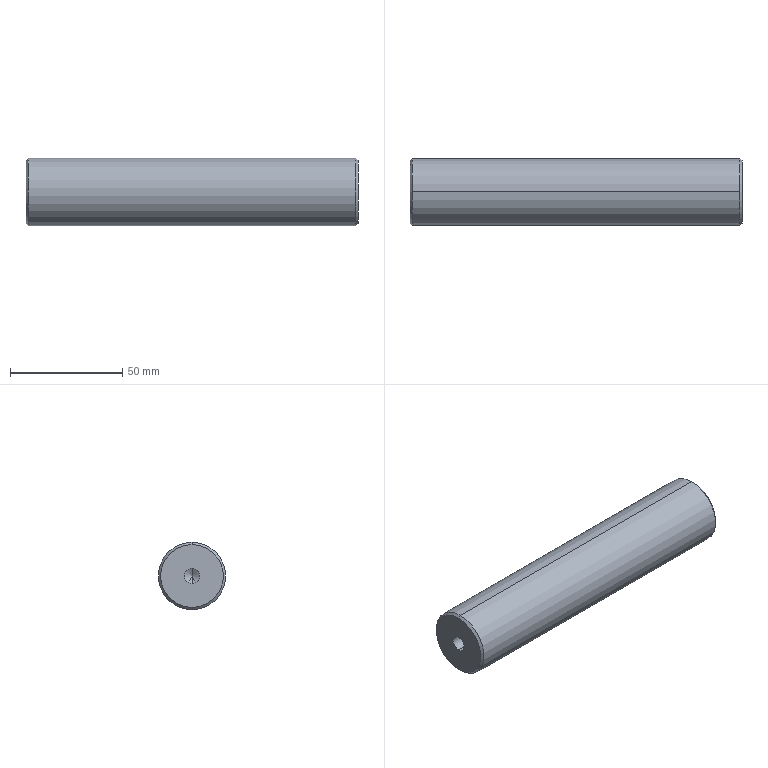Component | SolidWorks | GuideMechanism-1_ConnectingRod-1 | 1 solid | 16 faces | box 148 x 30 x 30 mm | volume 103039 mm3 | cone 8 | cylinder 6 | plane 2 | commonest cylinder face diameters 6.8 x4 30 x2
build123d program:
from build123d import *

# Parameters (mm, degrees)
SKETCH1_R           = 15
BOSS_EXTRUDE1_DEPTH = 74
CHAMFER1_SIZE       = 1


with BuildPart() as part:
    # Sketch1 → Boss-Extrude1 (new, symmetric)
    with BuildSketch(Plane(origin=(0, 0, 0), x_dir=(0, 0, -1), z_dir=(1, 0, 0))):
        Circle(SKETCH1_R)
    extrude(amount=BOSS_EXTRUDE1_DEPTH, both=True)

    # Sketch3 → M8 Tapped Hole1 (revolve, cut)
    with BuildSketch(Plane(origin=(74, 0, 0), x_dir=(0, 0, -1), z_dir=(0, 1, 0))):
        Polygon((0, 0), (0, 21.793), (3.4, 19.75), (3.4, 0), align=None)
    m8_tapped_hole1 = revolve(axis=Axis((80.35, 0, 0), (-1, 0, 0)), mode=Mode.SUBTRACT)

    # Mirror1: M8 Tapped Hole1 across plane
    add(m8_tapped_hole1.mirror(Plane(origin=(0, 0, 0), x_dir=(0, 0, 1), z_dir=(1, 0, 0))), mode=Mode.SUBTRACT)

    # Chamfer1
    chamfer1_edges = [part.edges().sort_by_distance(p)[0] for p in [
        (-74, 0, 15),
        (74, 0, 15),
    ]]
    chamfer(chamfer1_edges, length=CHAMFER1_SIZE)


solid = part.part

# Placed as in the assembly
solid = solid.moved(Location((-439.272, -518.766, 1326.5), (0, 0, 0)))
STEP:
#1=COLOUR_RGB('',0.7922,0.8196,0.9333);
#2=FILL_AREA_STYLE_COLOUR('',#1);
#3=FILL_AREA_STYLE('',(#2));
#4=SURFACE_STYLE_FILL_AREA(#3);
#5=SURFACE_SIDE_STYLE('',(#4));
#6=SURFACE_STYLE_USAGE(.BOTH.,#5);
#7=PRESENTATION_STYLE_ASSIGNMENT((#6));
#8=CARTESIAN_POINT('',(-20.208,-20.424,52.776));
#9=VERTEX_POINT('',#8);
#10=CARTESIAN_POINT('',(-20.208,-20.424,51.673));
#11=VERTEX_POINT('',#10);
#12=CARTESIAN_POINT('',(-20.208,-20.424,52.224));
#13=DIRECTION('',(-1.,0.,0.));
#14=DIRECTION('',(0.,0.,-1.));
#15=AXIS2_PLACEMENT_3D('',#12,#13,#14);
#16=CIRCLE('',#15,0.5512);
#17=EDGE_CURVE('',#9,#11,#16,.T.);
#18=ORIENTED_EDGE('',*,*,#17,.F.);
#19=CARTESIAN_POINT('',(-20.168,-20.424,52.815));
#20=VERTEX_POINT('',#19);
#21=CARTESIAN_POINT('',(-20.168,-20.424,52.815));
#22=DIRECTION('',(0.7071,0.,0.7071));
#23=VECTOR('',#22,39.37);
#24=LINE('',#21,#23);
#25=EDGE_CURVE('',#9,#20,#24,.T.);
#26=ORIENTED_EDGE('',*,*,#25,.T.);
#27=CARTESIAN_POINT('',(-20.168,-20.424,51.634));
#28=VERTEX_POINT('',#27);
#29=CARTESIAN_POINT('',(-20.168,-20.424,52.224));
#30=DIRECTION('',(1.,0.,0.));
#31=DIRECTION('',(0.,0.,-1.));
#32=AXIS2_PLACEMENT_3D('',#29,#30,#31);
#33=CIRCLE('',#32,0.5906);
#34=EDGE_CURVE('',#28,#20,#33,.T.);
#35=ORIENTED_EDGE('',*,*,#34,.F.);
#36=CARTESIAN_POINT('',(-20.168,-20.424,51.634));
#37=DIRECTION('',(0.7071,0.,-0.7071));
#38=VECTOR('',#37,39.37);
#39=LINE('',#36,#38);
#40=EDGE_CURVE('',#11,#28,#39,.T.);
#41=ORIENTED_EDGE('',*,*,#40,.F.);
#42=EDGE_LOOP('',(#18,#26,#35,#41));
#43=FACE_OUTER_BOUND('',#42,.T.);
#44=CARTESIAN_POINT('',(-20.168,-20.424,52.224));
#45=DIRECTION('',(1.,0.,0.));
#46=DIRECTION('',(0.,0.,-1.));
#47=AXIS2_PLACEMENT_3D('',#44,#45,#46);
#48=CONICAL_SURFACE('',#47,0.5906,0.7854);
#49=ADVANCED_FACE('',(#43),#48,.T.);
#50=CARTESIAN_POINT('',(-14.381,-20.424,51.673));
#51=VERTEX_POINT('',#50);
#52=CARTESIAN_POINT('',(-14.381,-20.424,52.776));
#53=VERTEX_POINT('',#52);
#54=CARTESIAN_POINT('',(-14.381,-20.424,52.224));
#55=DIRECTION('',(1.,0.,0.));
#56=DIRECTION('',(0.,0.,-1.));
#57=AXIS2_PLACEMENT_3D('',#54,#55,#56);
#58=CIRCLE('',#57,0.5512);
#59=EDGE_CURVE('',#51,#53,#58,.T.);
#60=ORIENTED_EDGE('',*,*,#59,.F.);
#61=CARTESIAN_POINT('',(-14.42,-20.424,51.634));
#62=VERTEX_POINT('',#61);
#63=CARTESIAN_POINT('',(-14.381,-20.424,51.673));
#64=DIRECTION('',(-0.7071,0.,-0.7071));
#65=VECTOR('',#64,39.37);
#66=LINE('',#63,#65);
#67=EDGE_CURVE('',#51,#62,#66,.T.);
#68=ORIENTED_EDGE('',*,*,#67,.T.);
#69=CARTESIAN_POINT('',(-14.42,-20.424,52.815));
#70=VERTEX_POINT('',#69);
#71=CARTESIAN_POINT('',(-14.42,-20.424,52.224));
#72=DIRECTION('',(-1.,0.,0.));
#73=DIRECTION('',(0.,0.,-1.));
#74=AXIS2_PLACEMENT_3D('',#71,#72,#73);
#75=CIRCLE('',#74,0.5906);
#76=EDGE_CURVE('',#70,#62,#75,.T.);
#77=ORIENTED_EDGE('',*,*,#76,.F.);
#78=CARTESIAN_POINT('',(-14.381,-20.424,52.776));
#79=DIRECTION('',(-0.7071,0.,0.7071));
#80=VECTOR('',#79,39.37);
#81=LINE('',#78,#80);
#82=EDGE_CURVE('',#53,#70,#81,.T.);
#83=ORIENTED_EDGE('',*,*,#82,.F.);
#84=EDGE_LOOP('',(#60,#68,#77,#83));
#85=FACE_OUTER_BOUND('',#84,.T.);
#86=CARTESIAN_POINT('',(-14.381,-20.424,52.224));
#87=DIRECTION('',(-1.,0.,0.));
#88=DIRECTION('',(0.,0.,1.));
#89=AXIS2_PLACEMENT_3D('',#86,#87,#88);
#90=CONICAL_SURFACE('',#89,0.5512,0.7854);
#91=ADVANCED_FACE('',(#85),#90,.T.);
#92=CARTESIAN_POINT('',(-19.43,-20.424,52.091));
#93=VERTEX_POINT('',#92);
#94=CARTESIAN_POINT('',(-19.43,-20.424,52.358));
#95=VERTEX_POINT('',#94);
#96=CARTESIAN_POINT('',(-19.43,-20.424,52.224));
#97=DIRECTION('',(-1.,0.,0.));
#98=DIRECTION('',(0.,0.,1.));
#99=AXIS2_PLACEMENT_3D('',#96,#97,#98);
#100=CIRCLE('',#99,0.1339);
#101=EDGE_CURVE('',#93,#95,#100,.T.);
#102=ORIENTED_EDGE('',*,*,#101,.F.);
#103=CARTESIAN_POINT('',(-20.208,-20.424,52.091));
#104=VERTEX_POINT('',#103);
#105=CARTESIAN_POINT('',(-20.208,-20.424,52.091));
#106=DIRECTION('',(-1.,0.,0.));
#107=VECTOR('',#106,39.37);
#108=LINE('',#105,#107);
#109=EDGE_CURVE('',#93,#104,#108,.T.);
#110=ORIENTED_EDGE('',*,*,#109,.T.);
#111=CARTESIAN_POINT('',(-20.208,-20.424,52.358));
#112=VERTEX_POINT('',#111);
#113=CARTESIAN_POINT('',(-20.208,-20.424,52.224));
#114=DIRECTION('',(-1.,0.,0.));
#115=DIRECTION('',(0.,0.,1.));
#116=AXIS2_PLACEMENT_3D('',#113,#114,#115);
#117=CIRCLE('',#116,0.1339);
#118=EDGE_CURVE('',#104,#112,#117,.T.);
#119=ORIENTED_EDGE('',*,*,#118,.T.);
#120=CARTESIAN_POINT('',(-20.208,-20.424,52.358));
#121=DIRECTION('',(-1.,0.,0.));
#122=VECTOR('',#121,39.37);
#123=LINE('',#120,#122);
#124=EDGE_CURVE('',#95,#112,#123,.T.);
#125=ORIENTED_EDGE('',*,*,#124,.F.);
#126=EDGE_LOOP('',(#102,#110,#119,#125));
#127=FACE_OUTER_BOUND('',#126,.T.);
#128=CARTESIAN_POINT('',(-20.208,-20.424,52.224));
#129=DIRECTION('',(-1.,0.,0.));
#130=DIRECTION('',(0.,0.,1.));
#131=AXIS2_PLACEMENT_3D('',#128,#129,#130);
#132=CYLINDRICAL_SURFACE('',#131,0.1339);
#133=ADVANCED_FACE('',(#127),#132,.F.);
#134=CARTESIAN_POINT('',(-19.35,-20.424,52.224));
#135=VERTEX_POINT('',#134);
#136=CARTESIAN_POINT('',(-19.43,-20.424,52.358));
#137=DIRECTION('',(-0.515,0.,0.8572));
#138=VECTOR('',#137,39.37);
#139=LINE('',#136,#138);
#140=EDGE_CURVE('',#135,#95,#139,.T.);
#141=ORIENTED_EDGE('',*,*,#140,.F.);
#142=CARTESIAN_POINT('',(-19.43,-20.424,52.091));
#143=DIRECTION('',(-0.515,0.,-0.8572));
#144=VECTOR('',#143,39.37);
#145=LINE('',#142,#144);
#146=EDGE_CURVE('',#135,#93,#145,.T.);
#147=ORIENTED_EDGE('',*,*,#146,.T.);
#148=ORIENTED_EDGE('',*,*,#101,.T.);
#149=EDGE_LOOP('',(#141,#147,#148));
#150=FACE_OUTER_BOUND('',#149,.T.);
#151=CARTESIAN_POINT('',(-19.43,-20.424,52.224));
#152=DIRECTION('',(-1.,0.,0.));
#153=DIRECTION('',(0.,0.,1.));
#154=AXIS2_PLACEMENT_3D('',#151,#152,#153);
#155=CONICAL_SURFACE('',#154,0.1339,1.03);
#156=ADVANCED_FACE('',(#150),#155,.F.);
#157=CARTESIAN_POINT('',(-15.158,-20.424,52.358));
#158=VERTEX_POINT('',#157);
#159=CARTESIAN_POINT('',(-15.158,-20.424,52.091));
#160=VERTEX_POINT('',#159);
#161=CARTESIAN_POINT('',(-15.158,-20.424,52.224));
#162=DIRECTION('',(1.,0.,0.));
#163=DIRECTION('',(0.,0.,-1.));
#164=AXIS2_PLACEMENT_3D('',#161,#162,#163);
#165=CIRCLE('',#164,0.1339);
#166=EDGE_CURVE('',#158,#160,#165,.T.);
#167=ORIENTED_EDGE('',*,*,#166,.F.);
#168=CARTESIAN_POINT('',(-14.381,-20.424,52.358));
#169=VERTEX_POINT('',#168);
#170=CARTESIAN_POINT('',(-14.381,-20.424,52.358));
#171=DIRECTION('',(1.,0.,0.));
#172=VECTOR('',#171,39.37);
#173=LINE('',#170,#172);
#174=EDGE_CURVE('',#158,#169,#173,.T.);
#175=ORIENTED_EDGE('',*,*,#174,.T.);
#176=CARTESIAN_POINT('',(-14.381,-20.424,52.091));
#177=VERTEX_POINT('',#176);
#178=CARTESIAN_POINT('',(-14.381,-20.424,52.224));
#179=DIRECTION('',(1.,0.,0.));
#180=DIRECTION('',(0.,0.,-1.));
#181=AXIS2_PLACEMENT_3D('',#178,#179,#180);
#182=CIRCLE('',#181,0.1339);
#183=EDGE_CURVE('',#169,#177,#182,.T.);
#184=ORIENTED_EDGE('',*,*,#183,.T.);
#185=CARTESIAN_POINT('',(-14.381,-20.424,52.091));
#186=DIRECTION('',(1.,0.,0.));
#187=VECTOR('',#186,39.37);
#188=LINE('',#185,#187);
#189=EDGE_CURVE('',#160,#177,#188,.T.);
#190=ORIENTED_EDGE('',*,*,#189,.F.);
#191=EDGE_LOOP('',(#167,#175,#184,#190));
#192=FACE_OUTER_BOUND('',#191,.T.);
#193=CARTESIAN_POINT('',(-14.381,-20.424,52.224));
#194=DIRECTION('',(1.,0.,0.));
#195=DIRECTION('',(0.,0.,-1.));
#196=AXIS2_PLACEMENT_3D('',#193,#194,#195);
#197=CYLINDRICAL_SURFACE('',#196,0.1339);
#198=ADVANCED_FACE('',(#192),#197,.F.);
#199=CARTESIAN_POINT('',(-15.239,-20.424,52.224));
#200=VERTEX_POINT('',#199);
#201=CARTESIAN_POINT('',(-15.158,-20.424,52.091));
#202=DIRECTION('',(0.515,0.,-0.8572));
#203=VECTOR('',#202,39.37);
#204=LINE('',#201,#203);
#205=EDGE_CURVE('',#200,#160,#204,.T.);
#206=ORIENTED_EDGE('',*,*,#205,.F.);
#207=CARTESIAN_POINT('',(-15.158,-20.424,52.358));
#208=DIRECTION('',(0.515,0.,0.8572));
#209=VECTOR('',#208,39.37);
#210=LINE('',#207,#209);
#211=EDGE_CURVE('',#200,#158,#210,.T.);
#212=ORIENTED_EDGE('',*,*,#211,.T.);
#213=ORIENTED_EDGE('',*,*,#166,.T.);
#214=EDGE_LOOP('',(#206,#212,#213));
#215=FACE_OUTER_BOUND('',#214,.T.);
#216=CARTESIAN_POINT('',(-15.158,-20.424,52.224));
#217=DIRECTION('',(1.,0.,0.));
#218=DIRECTION('',(0.,0.,-1.));
#219=AXIS2_PLACEMENT_3D('',#216,#217,#218);
#220=CONICAL_SURFACE('',#219,0.1339,1.03);
#221=ADVANCED_FACE('',(#215),#220,.F.);
#222=ORIENTED_EDGE('',*,*,#76,.T.);
#223=CARTESIAN_POINT('',(-14.381,-20.424,51.634));
#224=DIRECTION('',(-1.,0.,0.));
#225=VECTOR('',#224,39.37);
#226=LINE('',#223,#225);
#227=EDGE_CURVE('',#62,#28,#226,.T.);
#228=ORIENTED_EDGE('',*,*,#227,.T.);
#229=ORIENTED_EDGE('',*,*,#34,.T.);
#230=CARTESIAN_POINT('',(-14.381,-20.424,52.815));
#231=DIRECTION('',(-1.,0.,0.));
#232=VECTOR('',#231,39.37);
#233=LINE('',#230,#232);
#234=EDGE_CURVE('',#70,#20,#233,.T.);
#235=ORIENTED_EDGE('',*,*,#234,.F.);
#236=EDGE_LOOP('',(#222,#228,#229,#235));
#237=FACE_OUTER_BOUND('',#236,.T.);
#238=CARTESIAN_POINT('',(-14.381,-20.424,52.224));
#239=DIRECTION('',(-1.,0.,0.));
#240=DIRECTION('',(0.,0.,1.));
#241=AXIS2_PLACEMENT_3D('',#238,#239,#240);
#242=CYLINDRICAL_SURFACE('',#241,0.5906);
#243=ADVANCED_FACE('',(#237),#242,.T.);
#244=ORIENTED_EDGE('',*,*,#227,.F.);
#245=CARTESIAN_POINT('',(-14.42,-20.424,52.224));
#246=DIRECTION('',(-1.,0.,0.));
#247=DIRECTION('',(0.,0.,-1.));
#248=AXIS2_PLACEMENT_3D('',#245,#246,#247);
#249=CIRCLE('',#248,0.5906);
#250=EDGE_CURVE('',#62,#70,#249,.T.);
#251=ORIENTED_EDGE('',*,*,#250,.T.);
#252=ORIENTED_EDGE('',*,*,#234,.T.);
#253=CARTESIAN_POINT('',(-20.168,-20.424,52.224));
#254=DIRECTION('',(1.,0.,0.));
#255=DIRECTION('',(0.,0.,-1.));
#256=AXIS2_PLACEMENT_3D('',#253,#254,#255);
#257=CIRCLE('',#256,0.5906);
#258=EDGE_CURVE('',#20,#28,#257,.T.);
#259=ORIENTED_EDGE('',*,*,#258,.T.);
#260=EDGE_LOOP('',(#244,#251,#252,#259));
#261=FACE_OUTER_BOUND('',#260,.T.);
#262=CARTESIAN_POINT('',(-14.381,-20.424,52.224));
#263=DIRECTION('',(-1.,0.,0.));
#264=DIRECTION('',(0.,0.,1.));
#265=AXIS2_PLACEMENT_3D('',#262,#263,#264);
#266=CYLINDRICAL_SURFACE('',#265,0.5906);
#267=ADVANCED_FACE('',(#261),#266,.T.);
#268=CARTESIAN_POINT('',(-14.381,-20.424,52.224));
#269=DIRECTION('',(1.,0.,0.));
#270=DIRECTION('',(0.,0.,-1.));
#271=AXIS2_PLACEMENT_3D('',#268,#269,#270);
#272=CIRCLE('',#271,0.5512);
#273=EDGE_CURVE('',#53,#51,#272,.T.);
#274=ORIENTED_EDGE('',*,*,#273,.T.);
#275=ORIENTED_EDGE('',*,*,#59,.T.);
#276=EDGE_LOOP('',(#274,#275));
#277=FACE_OUTER_BOUND('',#276,.T.);
#278=CARTESIAN_POINT('',(-14.381,-20.424,52.224));
#279=DIRECTION('',(1.,0.,0.));
#280=DIRECTION('',(0.,0.,-1.));
#281=AXIS2_PLACEMENT_3D('',#278,#279,#280);
#282=CIRCLE('',#281,0.1339);
#283=EDGE_CURVE('',#177,#169,#282,.T.);
#284=ORIENTED_EDGE('',*,*,#283,.F.);
#285=ORIENTED_EDGE('',*,*,#183,.F.);
#286=EDGE_LOOP('',(#284,#285));
#287=FACE_BOUND('',#286,.T.);
#288=CARTESIAN_POINT('',(-14.381,-20.424,52.224));
#289=DIRECTION('',(1.,0.,0.));
#290=DIRECTION('',(0.,0.,-1.));
#291=AXIS2_PLACEMENT_3D('',#288,#289,#290);
#292=PLANE('',#291);
#293=ADVANCED_FACE('',(#277,#287),#292,.T.);
#294=CARTESIAN_POINT('',(-20.208,-20.424,52.224));
#295=DIRECTION('',(-1.,0.,0.));
#296=DIRECTION('',(0.,0.,-1.));
#297=AXIS2_PLACEMENT_3D('',#294,#295,#296);
#298=CIRCLE('',#297,0.5512);
#299=EDGE_CURVE('',#11,#9,#298,.T.);
#300=ORIENTED_EDGE('',*,*,#299,.T.);
#301=ORIENTED_EDGE('',*,*,#17,.T.);
#302=EDGE_LOOP('',(#300,#301));
#303=FACE_OUTER_BOUND('',#302,.T.);
#304=CARTESIAN_POINT('',(-20.208,-20.424,52.224));
#305=DIRECTION('',(-1.,0.,0.));
#306=DIRECTION('',(0.,0.,1.));
#307=AXIS2_PLACEMENT_3D('',#304,#305,#306);
#308=CIRCLE('',#307,0.1339);
#309=EDGE_CURVE('',#112,#104,#308,.T.);
#310=ORIENTED_EDGE('',*,*,#309,.F.);
#311=ORIENTED_EDGE('',*,*,#118,.F.);
#312=EDGE_LOOP('',(#310,#311));
#313=FACE_BOUND('',#312,.T.);
#314=CARTESIAN_POINT('',(-20.208,-20.424,52.224));
#315=DIRECTION('',(1.,0.,0.));
#316=DIRECTION('',(0.,0.,-1.));
#317=AXIS2_PLACEMENT_3D('',#314,#315,#316);
#318=PLANE('',#317);
#319=ADVANCED_FACE('',(#303,#313),#318,.F.);
#320=ORIENTED_EDGE('',*,*,#211,.F.);
#321=ORIENTED_EDGE('',*,*,#205,.T.);
#322=CARTESIAN_POINT('',(-15.158,-20.424,52.224));
#323=DIRECTION('',(1.,0.,0.));
#324=DIRECTION('',(0.,0.,-1.));
#325=AXIS2_PLACEMENT_3D('',#322,#323,#324);
#326=CIRCLE('',#325,0.1339);
#327=EDGE_CURVE('',#160,#158,#326,.T.);
#328=ORIENTED_EDGE('',*,*,#327,.T.);
#329=EDGE_LOOP('',(#320,#321,#328));
#330=FACE_OUTER_BOUND('',#329,.T.);
#331=CARTESIAN_POINT('',(-15.158,-20.424,52.224));
#332=DIRECTION('',(1.,0.,0.));
#333=DIRECTION('',(0.,0.,-1.));
#334=AXIS2_PLACEMENT_3D('',#331,#332,#333);
#335=CONICAL_SURFACE('',#334,0.1339,1.03);
#336=ADVANCED_FACE('',(#330),#335,.F.);
#337=ORIENTED_EDGE('',*,*,#174,.F.);
#338=ORIENTED_EDGE('',*,*,#327,.F.);
#339=ORIENTED_EDGE('',*,*,#189,.T.);
#340=ORIENTED_EDGE('',*,*,#283,.T.);
#341=EDGE_LOOP('',(#337,#338,#339,#340));
#342=FACE_OUTER_BOUND('',#341,.T.);
#343=CARTESIAN_POINT('',(-14.381,-20.424,52.224));
#344=DIRECTION('',(1.,0.,0.));
#345=DIRECTION('',(0.,0.,-1.));
#346=AXIS2_PLACEMENT_3D('',#343,#344,#345);
#347=CYLINDRICAL_SURFACE('',#346,0.1339);
#348=ADVANCED_FACE('',(#342),#347,.F.);
#349=ORIENTED_EDGE('',*,*,#146,.F.);
#350=ORIENTED_EDGE('',*,*,#140,.T.);
#351=CARTESIAN_POINT('',(-19.43,-20.424,52.224));
#352=DIRECTION('',(-1.,0.,0.));
#353=DIRECTION('',(0.,0.,1.));
#354=AXIS2_PLACEMENT_3D('',#351,#352,#353);
#355=CIRCLE('',#354,0.1339);
#356=EDGE_CURVE('',#95,#93,#355,.T.);
#357=ORIENTED_EDGE('',*,*,#356,.T.);
#358=EDGE_LOOP('',(#349,#350,#357));
#359=FACE_OUTER_BOUND('',#358,.T.);
#360=CARTESIAN_POINT('',(-19.43,-20.424,52.224));
#361=DIRECTION('',(-1.,0.,0.));
#362=DIRECTION('',(0.,0.,1.));
#363=AXIS2_PLACEMENT_3D('',#360,#361,#362);
#364=CONICAL_SURFACE('',#363,0.1339,1.03);
#365=ADVANCED_FACE('',(#359),#364,.F.);
#366=ORIENTED_EDGE('',*,*,#109,.F.);
#367=ORIENTED_EDGE('',*,*,#356,.F.);
#368=ORIENTED_EDGE('',*,*,#124,.T.);
#369=ORIENTED_EDGE('',*,*,#309,.T.);
#370=EDGE_LOOP('',(#366,#367,#368,#369));
#371=FACE_OUTER_BOUND('',#370,.T.);
#372=CARTESIAN_POINT('',(-20.208,-20.424,52.224));
#373=DIRECTION('',(-1.,0.,0.));
#374=DIRECTION('',(0.,0.,1.));
#375=AXIS2_PLACEMENT_3D('',#372,#373,#374);
#376=CYLINDRICAL_SURFACE('',#375,0.1339);
#377=ADVANCED_FACE('',(#371),#376,.F.);
#378=ORIENTED_EDGE('',*,*,#67,.F.);
#379=ORIENTED_EDGE('',*,*,#273,.F.);
#380=ORIENTED_EDGE('',*,*,#82,.T.);
#381=ORIENTED_EDGE('',*,*,#250,.F.);
#382=EDGE_LOOP('',(#378,#379,#380,#381));
#383=FACE_OUTER_BOUND('',#382,.T.);
#384=CARTESIAN_POINT('',(-14.381,-20.424,52.224));
#385=DIRECTION('',(-1.,0.,0.));
#386=DIRECTION('',(0.,0.,1.));
#387=AXIS2_PLACEMENT_3D('',#384,#385,#386);
#388=CONICAL_SURFACE('',#387,0.5512,0.7854);
#389=ADVANCED_FACE('',(#383),#388,.T.);
#390=ORIENTED_EDGE('',*,*,#25,.F.);
#391=ORIENTED_EDGE('',*,*,#299,.F.);
#392=ORIENTED_EDGE('',*,*,#40,.T.);
#393=ORIENTED_EDGE('',*,*,#258,.F.);
#394=EDGE_LOOP('',(#390,#391,#392,#393));
#395=FACE_OUTER_BOUND('',#394,.T.);
#396=CARTESIAN_POINT('',(-20.168,-20.424,52.224));
#397=DIRECTION('',(1.,0.,0.));
#398=DIRECTION('',(0.,0.,-1.));
#399=AXIS2_PLACEMENT_3D('',#396,#397,#398);
#400=CONICAL_SURFACE('',#399,0.5906,0.7854);
#401=ADVANCED_FACE('',(#395),#400,.T.);
#402=CLOSED_SHELL('',(#49,#91,#133,#156,#198,#221,#243,#267,#293,#319,#336,#348,#365,#377,#389,#401));
#403=MANIFOLD_SOLID_BREP('',#402);
#404=STYLED_ITEM('',(#7),#403);
#405=PRESENTATION_LAYER_ASSIGNMENT('','',(#404));
#406=CARTESIAN_POINT('',(0.,0.,0.));
#407=DIRECTION('',(0.,0.,1.));
#408=DIRECTION('',(1.,0.,0.));
#409=AXIS2_PLACEMENT_3D('',#406,#407,#408);
#410=(LENGTH_UNIT()NAMED_UNIT(*)SI_UNIT($,.METRE.));
#411=LENGTH_MEASURE_WITH_UNIT(LENGTH_MEASURE(0.0254),#410);
#412=DIMENSIONAL_EXPONENTS(1.,0.,0.,0.,0.,0.,0.);
#413=(CONVERSION_BASED_UNIT('',#411)LENGTH_UNIT()NAMED_UNIT(#412));
#414=UNCERTAINTY_MEASURE_WITH_UNIT(LENGTH_MEASURE(0.00001),#413,'','');
#415=(NAMED_UNIT(*)PLANE_ANGLE_UNIT()SI_UNIT($,.RADIAN.));
#416=(NAMED_UNIT(*)SI_UNIT($,.STERADIAN.)SOLID_ANGLE_UNIT());
#417=(GEOMETRIC_REPRESENTATION_CONTEXT(3)GLOBAL_UNCERTAINTY_ASSIGNED_CONTEXT((#414))GLOBAL_UNIT_ASSIGNED_CONTEXT((#413,#415,#416))REPRESENTATION_CONTEXT('',''));
#418=ADVANCED_BREP_SHAPE_REPRESENTATION('',(#403,#409),#417);
#419=(LENGTH_UNIT()NAMED_UNIT(*)SI_UNIT($,.METRE.));
#420=LENGTH_MEASURE_WITH_UNIT(LENGTH_MEASURE(0.0254),#419);
#421=DIMENSIONAL_EXPONENTS(1.,0.,0.,0.,0.,0.,0.);
#422=(CONVERSION_BASED_UNIT('',#420)LENGTH_UNIT()NAMED_UNIT(#421));
#423=UNCERTAINTY_MEASURE_WITH_UNIT(LENGTH_MEASURE(0.00001),#422,'','');
#424=(NAMED_UNIT(*)PLANE_ANGLE_UNIT()SI_UNIT($,.RADIAN.));
#425=(NAMED_UNIT(*)SI_UNIT($,.STERADIAN.)SOLID_ANGLE_UNIT());
#426=(GEOMETRIC_REPRESENTATION_CONTEXT(3)GLOBAL_UNCERTAINTY_ASSIGNED_CONTEXT((#423))GLOBAL_UNIT_ASSIGNED_CONTEXT((#422,#424,#425))REPRESENTATION_CONTEXT('',''));
#427=MECHANICAL_DESIGN_GEOMETRIC_PRESENTATION_REPRESENTATION('',(#404),#426);